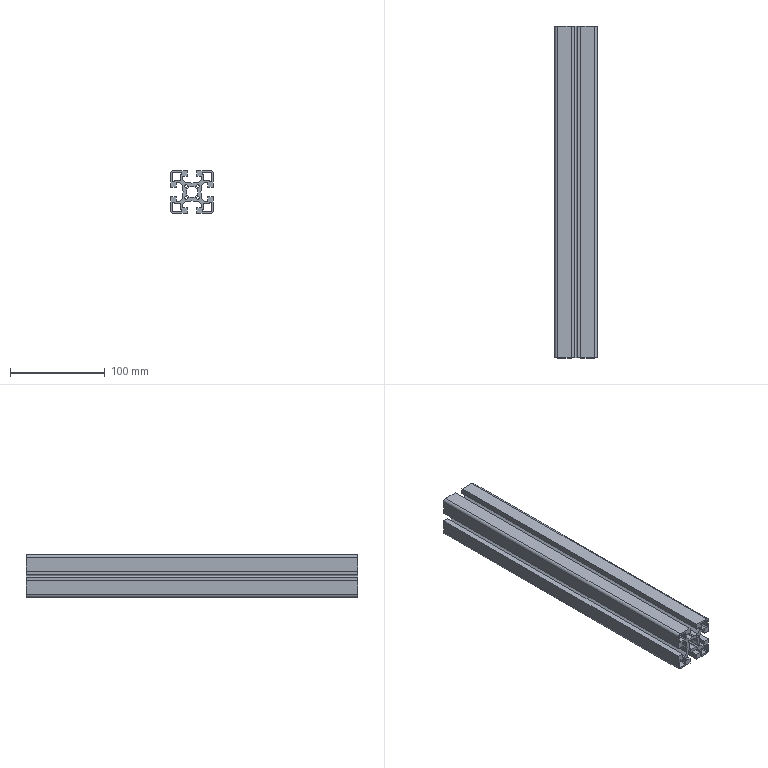Component | SolidWorks | HFS8_4545_07-B-3 | 1 solid | 131 faces | box 45 x 350 x 45 mm | volume 280770 mm3 | plane 82 | cylinder 49 | commonest cylinder face diameters 2 x18 3 x12 1 x10 12.5 x5 6 x4
build123d program:
from build123d import *

# Parameters (mm, degrees)
BOSS_EXTRUDE1_DEPTH = 350


with BuildPart() as part:
    # Sketch1 → Boss-Extrude1 (new body)
    with BuildSketch(Plane.XY):
        with BuildLine():
            Line((-19.5, -22.5), (-5, -22.5))
            Line((-5, -22.5), (-5, -16.5))
            Line((-5, -16.5), (-10, -16.5))
            Line((-10, -16.5), (-10, -13))
            Line((-10, -13), (-6.5, -9.5))
            Line((-6.5, -9.5), (-1.212, -9.5))
            Line((-1.212, -9.5), (0, -8.8))
            Line((0, -8.8), (1.212, -9.5))
            Line((1.212, -9.5), (6.5, -9.5))
            Line((6.5, -9.5), (10, -13))
            Line((10, -13), (10, -16.5))
            Line((10, -16.5), (5, -16.5))
            Line((5, -16.5), (5, -22.5))
            Line((5, -22.5), (19.5, -22.5))
            ThreePointArc((19.5, -22.5), (21.621, -21.621), (22.5, -19.5))
            Line((22.5, -19.5), (22.5, -5))
            Line((22.5, -5), (16.5, -5))
            Line((16.5, -5), (16.5, -10))
            Line((16.5, -10), (13, -10))
            Line((13, -10), (9.5, -6.5))
            Line((9.5, -6.5), (9.5, -1.212))
            Line((9.5, -1.212), (8.8, 0))
            Line((8.8, 0), (9.5, 1.212))
            Line((9.5, 1.212), (9.5, 6.5))
            Line((9.5, 6.5), (13, 10))
            Line((13, 10), (16.5, 10))
            Line((16.5, 10), (16.5, 5))
            Line((16.5, 5), (22.5, 5))
            Line((22.5, 5), (22.5, 19.5))
            ThreePointArc((22.5, 19.5), (21.621, 21.621), (19.5, 22.5))
            Line((19.5, 22.5), (5, 22.5))
            Line((5, 22.5), (5, 16.5))
            Line((5, 16.5), (10, 16.5))
            Line((10, 16.5), (10, 13))
            Line((10, 13), (6.5, 9.5))
            Line((6.5, 9.5), (1.212, 9.5))
            Line((1.212, 9.5), (0, 8.8))
            Line((0, 8.8), (-1.212, 9.5))
            Line((-1.212, 9.5), (-6.5, 9.5))
            Line((-6.5, 9.5), (-10, 13))
            Line((-10, 13), (-10, 16.5))
            Line((-10, 16.5), (-5, 16.5))
            Line((-5, 16.5), (-5, 22.5))
            Line((-5, 22.5), (-19.5, 22.5))
            ThreePointArc((-19.5, 22.5), (-21.621, 21.621), (-22.5, 19.5))
            Line((-22.5, 19.5), (-22.5, 5))
            Line((-22.5, 5), (-16.5, 5))
            Line((-16.5, 5), (-16.5, 10))
            Line((-16.5, 10), (-13, 10))
            Line((-13, 10), (-9.5, 6.5))
            Line((-9.5, 6.5), (-9.5, 1.212))
            Line((-9.5, 1.212), (-8.8, 0))
            Line((-8.8, 0), (-9.5, -1.212))
            Line((-9.5, -1.212), (-9.5, -6.5))
            Line((-9.5, -6.5), (-13, -10))
            Line((-13, -10), (-16.5, -10))
            Line((-16.5, -10), (-16.5, -5))
            Line((-16.5, -5), (-22.5, -5))
            Line((-22.5, -5), (-22.5, -19.5))
            ThreePointArc((-22.5, -19.5), (-21.621, -21.621), (-19.5, -22.5))
        make_face()
        with BuildLine():
            Line((12, 18.5), (12, 13))
            ThreePointArc((12, 13), (12.293, 12.293), (13, 12))
            Line((13, 12), (18.5, 12))
            ThreePointArc((18.5, 12), (19.5, 11), (20.5, 12))
            Line((20.5, 12), (20.5, 19.5))
            ThreePointArc((20.5, 19.5), (20.207, 20.207), (19.5, 20.5))
            Line((19.5, 20.5), (12, 20.5))
            ThreePointArc((12, 20.5), (11, 19.5), (12, 18.5))
        make_face(mode=Mode.SUBTRACT)
        with BuildLine():
            Line((12, -20.5), (19.5, -20.5))
            ThreePointArc((19.5, -20.5), (20.207, -20.207), (20.5, -19.5))
            Line((20.5, -19.5), (20.5, -12))
            ThreePointArc((20.5, -12), (19.5, -11), (18.5, -12))
            Line((18.5, -12), (13, -12))
            ThreePointArc((13, -12), (12.293, -12.293), (12, -13))
            Line((12, -13), (12, -18.5))
            ThreePointArc((12, -18.5), (11, -19.5), (12, -20.5))
        make_face(mode=Mode.SUBTRACT)
        with BuildLine():
            Line((-4.725, -6.139), (-3.947, -5.361))
            ThreePointArc((-3.947, -5.361), (-3.649, -5.217), (-3.327, -5.291))
            ThreePointArc((-3.327, -5.291), (0, -6.25), (3.327, -5.291))
            ThreePointArc((3.327, -5.291), (3.649, -5.217), (3.947, -5.361))
            Line((3.947, -5.361), (4.725, -6.139))
            ThreePointArc((4.725, -6.139), (7.283, -7.283), (6.139, -4.725))
            Line((6.139, -4.725), (5.361, -3.947))
            ThreePointArc((5.361, -3.947), (5.217, -3.649), (5.291, -3.327))
            ThreePointArc((5.291, -3.327), (6.25, 0), (5.291, 3.327))
            ThreePointArc((5.291, 3.327), (5.217, 3.649), (5.361, 3.947))
            Line((5.361, 3.947), (6.139, 4.725))
            ThreePointArc((6.139, 4.725), (7.283, 7.283), (4.725, 6.139))
            Line((4.725, 6.139), (3.947, 5.361))
            ThreePointArc((3.947, 5.361), (3.649, 5.217), (3.327, 5.291))
            ThreePointArc((3.327, 5.291), (0, 6.25), (-3.327, 5.291))
            ThreePointArc((-3.327, 5.291), (-3.649, 5.217), (-3.947, 5.361))
            Line((-3.947, 5.361), (-4.725, 6.139))
            ThreePointArc((-4.725, 6.139), (-7.283, 7.283), (-6.139, 4.725))
            Line((-6.139, 4.725), (-5.361, 3.947))
            ThreePointArc((-5.361, 3.947), (-5.217, 3.649), (-5.291, 3.327))
            ThreePointArc((-5.291, 3.327), (-6.25, 0), (-5.291, -3.327))
            ThreePointArc((-5.291, -3.327), (-5.217, -3.649), (-5.361, -3.947))
            Line((-5.361, -3.947), (-6.139, -4.725))
            ThreePointArc((-6.139, -4.725), (-7.283, -7.283), (-4.725, -6.139))
        make_face(mode=Mode.SUBTRACT)
        with BuildLine():
            Line((-19.5, -20.5), (-12, -20.5))
            ThreePointArc((-12, -20.5), (-11, -19.5), (-12, -18.5))
            Line((-12, -18.5), (-12, -13))
            ThreePointArc((-12, -13), (-12.293, -12.293), (-13, -12))
            Line((-13, -12), (-18.5, -12))
            ThreePointArc((-18.5, -12), (-19.5, -11), (-20.5, -12))
            Line((-20.5, -12), (-20.5, -19.5))
            ThreePointArc((-20.5, -19.5), (-20.207, -20.207), (-19.5, -20.5))
        make_face(mode=Mode.SUBTRACT)
        with BuildLine():
            Line((-18.5, 12), (-13, 12))
            ThreePointArc((-13, 12), (-12.293, 12.293), (-12, 13))
            Line((-12, 13), (-12, 18.5))
            ThreePointArc((-12, 18.5), (-11, 19.5), (-12, 20.5))
            Line((-12, 20.5), (-19.5, 20.5))
            ThreePointArc((-19.5, 20.5), (-20.207, 20.207), (-20.5, 19.5))
            Line((-20.5, 19.5), (-20.5, 12))
            ThreePointArc((-20.5, 12), (-19.5, 11), (-18.5, 12))
        make_face(mode=Mode.SUBTRACT)
    extrude(amount=-BOSS_EXTRUDE1_DEPTH)


solid = part.part

# Placed as in the assembly
solid = solid.moved(Location((-820.506, -724.413, -970.428), (90, 0, 0)))